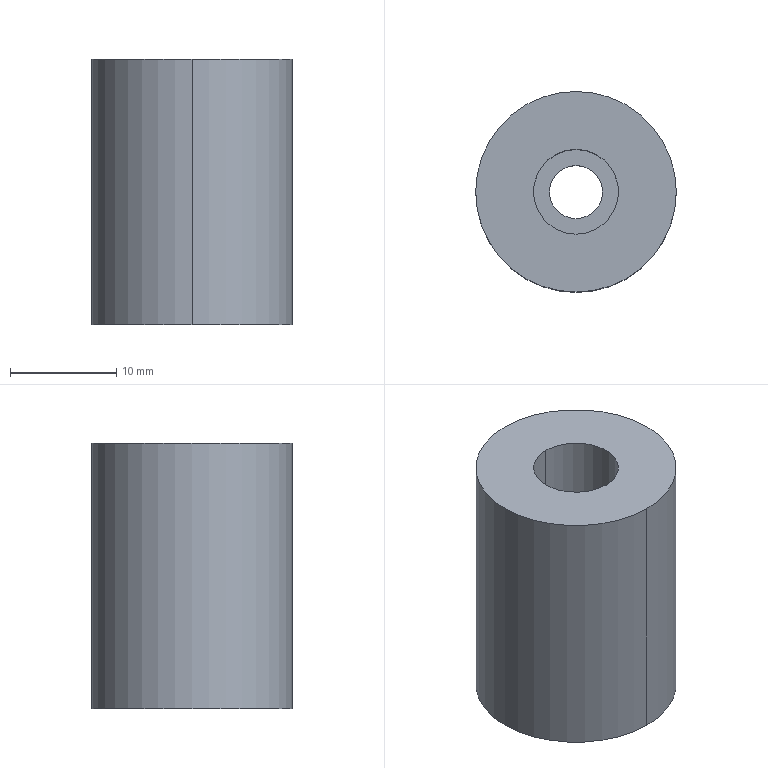Component | SolidWorks | Coupling2-1 | 1 solid | 9 faces | box 18.9 x 18.9 x 25 mm | volume 6033 mm3 | cylinder 6 | plane 3 | commonest cylinder face diameters 18.9 x2 8 x2 5 x2
STEP:
#1=COLOUR_RGB('',0.7922,0.8196,0.9333);
#2=FILL_AREA_STYLE_COLOUR('',#1);
#3=FILL_AREA_STYLE('',(#2));
#4=SURFACE_STYLE_FILL_AREA(#3);
#5=SURFACE_SIDE_STYLE('',(#4));
#6=SURFACE_STYLE_USAGE(.BOTH.,#5);
#7=PRESENTATION_STYLE_ASSIGNMENT((#6));
#8=CARTESIAN_POINT('',(0.,0.372,0.5315));
#9=VERTEX_POINT('',#8);
#10=CARTESIAN_POINT('',(-0.,-0.372,0.5315));
#11=VERTEX_POINT('',#10);
#12=CARTESIAN_POINT('',(0.,0.,0.5315));
#13=DIRECTION('',(-0.,-0.,1.));
#14=DIRECTION('',(-0.,1.,0.));
#15=AXIS2_PLACEMENT_3D('',#12,#13,#14);
#16=CIRCLE('',#15,0.372);
#17=EDGE_CURVE('',#9,#11,#16,.T.);
#18=ORIENTED_EDGE('',*,*,#17,.T.);
#19=CARTESIAN_POINT('',(-0.,-0.372,1.516));
#20=VERTEX_POINT('',#19);
#21=CARTESIAN_POINT('',(0.,-0.372,0.5315));
#22=DIRECTION('',(-0.,-0.,1.));
#23=VECTOR('',#22,39.37);
#24=LINE('',#21,#23);
#25=EDGE_CURVE('',#11,#20,#24,.T.);
#26=ORIENTED_EDGE('',*,*,#25,.T.);
#27=CARTESIAN_POINT('',(-0.,0.372,1.516));
#28=VERTEX_POINT('',#27);
#29=CARTESIAN_POINT('',(-0.,-0.,1.516));
#30=DIRECTION('',(0.,0.,-1.));
#31=DIRECTION('',(-0.,1.,0.));
#32=AXIS2_PLACEMENT_3D('',#29,#30,#31);
#33=CIRCLE('',#32,0.372);
#34=EDGE_CURVE('',#20,#28,#33,.T.);
#35=ORIENTED_EDGE('',*,*,#34,.T.);
#36=CARTESIAN_POINT('',(0.,0.372,0.5315));
#37=DIRECTION('',(-0.,-0.,1.));
#38=VECTOR('',#37,39.37);
#39=LINE('',#36,#38);
#40=EDGE_CURVE('',#9,#28,#39,.T.);
#41=ORIENTED_EDGE('',*,*,#40,.F.);
#42=EDGE_LOOP('',(#18,#26,#35,#41));
#43=FACE_OUTER_BOUND('',#42,.T.);
#44=CARTESIAN_POINT('',(0.,0.,0.5315));
#45=DIRECTION('',(-0.,-0.,1.));
#46=DIRECTION('',(-0.,1.,0.));
#47=AXIS2_PLACEMENT_3D('',#44,#45,#46);
#48=CYLINDRICAL_SURFACE('',#47,0.372);
#49=ADVANCED_FACE('',(#43),#48,.T.);
#50=CARTESIAN_POINT('',(-0.,-0.1575,0.8858));
#51=VERTEX_POINT('',#50);
#52=CARTESIAN_POINT('',(-0.,0.1575,0.8858));
#53=VERTEX_POINT('',#52);
#54=CARTESIAN_POINT('',(-0.,0.,0.8858));
#55=DIRECTION('',(-0.,-0.,1.));
#56=DIRECTION('',(-0.,1.,0.));
#57=AXIS2_PLACEMENT_3D('',#54,#55,#56);
#58=CIRCLE('',#57,0.1575);
#59=EDGE_CURVE('',#51,#53,#58,.T.);
#60=ORIENTED_EDGE('',*,*,#59,.F.);
#61=CARTESIAN_POINT('',(-0.,-0.1575,1.516));
#62=VERTEX_POINT('',#61);
#63=CARTESIAN_POINT('',(-0.,-0.1575,0.8858));
#64=DIRECTION('',(-0.,-0.,1.));
#65=VECTOR('',#64,39.37);
#66=LINE('',#63,#65);
#67=EDGE_CURVE('',#51,#62,#66,.T.);
#68=ORIENTED_EDGE('',*,*,#67,.T.);
#69=CARTESIAN_POINT('',(-0.,0.1575,1.516));
#70=VERTEX_POINT('',#69);
#71=CARTESIAN_POINT('',(-0.,-0.,1.516));
#72=DIRECTION('',(-0.,-0.,1.));
#73=DIRECTION('',(-0.,1.,0.));
#74=AXIS2_PLACEMENT_3D('',#71,#72,#73);
#75=CIRCLE('',#74,0.1575);
#76=EDGE_CURVE('',#62,#70,#75,.T.);
#77=ORIENTED_EDGE('',*,*,#76,.T.);
#78=CARTESIAN_POINT('',(-0.,0.1575,0.8858));
#79=DIRECTION('',(-0.,-0.,1.));
#80=VECTOR('',#79,39.37);
#81=LINE('',#78,#80);
#82=EDGE_CURVE('',#53,#70,#81,.T.);
#83=ORIENTED_EDGE('',*,*,#82,.F.);
#84=EDGE_LOOP('',(#60,#68,#77,#83));
#85=FACE_OUTER_BOUND('',#84,.T.);
#86=CARTESIAN_POINT('',(-0.,0.,0.8858));
#87=DIRECTION('',(-0.,-0.,1.));
#88=DIRECTION('',(-0.,1.,0.));
#89=AXIS2_PLACEMENT_3D('',#86,#87,#88);
#90=CYLINDRICAL_SURFACE('',#89,0.1575);
#91=ADVANCED_FACE('',(#85),#90,.F.);
#92=CARTESIAN_POINT('',(0.,-0.09843,0.5315));
#93=VERTEX_POINT('',#92);
#94=CARTESIAN_POINT('',(0.,0.09843,0.5315));
#95=VERTEX_POINT('',#94);
#96=CARTESIAN_POINT('',(0.,0.,0.5315));
#97=DIRECTION('',(-0.,-0.,1.));
#98=DIRECTION('',(-0.,1.,0.));
#99=AXIS2_PLACEMENT_3D('',#96,#97,#98);
#100=CIRCLE('',#99,0.09843);
#101=EDGE_CURVE('',#93,#95,#100,.T.);
#102=ORIENTED_EDGE('',*,*,#101,.F.);
#103=CARTESIAN_POINT('',(0.,-0.09843,0.8858));
#104=VERTEX_POINT('',#103);
#105=CARTESIAN_POINT('',(0.,-0.09843,0.2559));
#106=DIRECTION('',(-0.,-0.,1.));
#107=VECTOR('',#106,39.37);
#108=LINE('',#105,#107);
#109=EDGE_CURVE('',#93,#104,#108,.T.);
#110=ORIENTED_EDGE('',*,*,#109,.T.);
#111=CARTESIAN_POINT('',(-0.,0.09843,0.8858));
#112=VERTEX_POINT('',#111);
#113=CARTESIAN_POINT('',(-0.,0.,0.8858));
#114=DIRECTION('',(0.,0.,-1.));
#115=DIRECTION('',(-0.,1.,0.));
#116=AXIS2_PLACEMENT_3D('',#113,#114,#115);
#117=CIRCLE('',#116,0.09843);
#118=EDGE_CURVE('',#112,#104,#117,.T.);
#119=ORIENTED_EDGE('',*,*,#118,.F.);
#120=CARTESIAN_POINT('',(0.,0.09843,0.2559));
#121=DIRECTION('',(-0.,-0.,1.));
#122=VECTOR('',#121,39.37);
#123=LINE('',#120,#122);
#124=EDGE_CURVE('',#95,#112,#123,.T.);
#125=ORIENTED_EDGE('',*,*,#124,.F.);
#126=EDGE_LOOP('',(#102,#110,#119,#125));
#127=FACE_OUTER_BOUND('',#126,.T.);
#128=CARTESIAN_POINT('',(0.,0.,0.2559));
#129=DIRECTION('',(-0.,-0.,1.));
#130=DIRECTION('',(-0.,1.,0.));
#131=AXIS2_PLACEMENT_3D('',#128,#129,#130);
#132=CYLINDRICAL_SURFACE('',#131,0.09843);
#133=ADVANCED_FACE('',(#127),#132,.F.);
#134=ORIENTED_EDGE('',*,*,#25,.F.);
#135=CARTESIAN_POINT('',(0.,0.,0.5315));
#136=DIRECTION('',(-0.,-0.,1.));
#137=DIRECTION('',(-0.,1.,0.));
#138=AXIS2_PLACEMENT_3D('',#135,#136,#137);
#139=CIRCLE('',#138,0.372);
#140=EDGE_CURVE('',#11,#9,#139,.T.);
#141=ORIENTED_EDGE('',*,*,#140,.T.);
#142=ORIENTED_EDGE('',*,*,#40,.T.);
#143=CARTESIAN_POINT('',(-0.,-0.,1.516));
#144=DIRECTION('',(0.,0.,-1.));
#145=DIRECTION('',(-0.,1.,0.));
#146=AXIS2_PLACEMENT_3D('',#143,#144,#145);
#147=CIRCLE('',#146,0.372);
#148=EDGE_CURVE('',#28,#20,#147,.T.);
#149=ORIENTED_EDGE('',*,*,#148,.T.);
#150=EDGE_LOOP('',(#134,#141,#142,#149));
#151=FACE_OUTER_BOUND('',#150,.T.);
#152=CARTESIAN_POINT('',(0.,0.,0.5315));
#153=DIRECTION('',(-0.,-0.,1.));
#154=DIRECTION('',(-0.,1.,0.));
#155=AXIS2_PLACEMENT_3D('',#152,#153,#154);
#156=CYLINDRICAL_SURFACE('',#155,0.372);
#157=ADVANCED_FACE('',(#151),#156,.T.);
#158=ORIENTED_EDGE('',*,*,#148,.F.);
#159=ORIENTED_EDGE('',*,*,#34,.F.);
#160=EDGE_LOOP('',(#158,#159));
#161=FACE_OUTER_BOUND('',#160,.T.);
#162=CARTESIAN_POINT('',(-0.,-0.,1.516));
#163=DIRECTION('',(-0.,-0.,1.));
#164=DIRECTION('',(-0.,1.,0.));
#165=AXIS2_PLACEMENT_3D('',#162,#163,#164);
#166=CIRCLE('',#165,0.1575);
#167=EDGE_CURVE('',#70,#62,#166,.T.);
#168=ORIENTED_EDGE('',*,*,#167,.F.);
#169=ORIENTED_EDGE('',*,*,#76,.F.);
#170=EDGE_LOOP('',(#168,#169));
#171=FACE_BOUND('',#170,.T.);
#172=CARTESIAN_POINT('',(-0.,-0.,1.516));
#173=DIRECTION('',(0.,0.,-1.));
#174=DIRECTION('',(0.,-1.,-0.));
#175=AXIS2_PLACEMENT_3D('',#172,#173,#174);
#176=PLANE('',#175);
#177=ADVANCED_FACE('',(#161,#171),#176,.F.);
#178=ORIENTED_EDGE('',*,*,#17,.F.);
#179=ORIENTED_EDGE('',*,*,#140,.F.);
#180=EDGE_LOOP('',(#178,#179));
#181=FACE_OUTER_BOUND('',#180,.T.);
#182=CARTESIAN_POINT('',(0.,0.,0.5315));
#183=DIRECTION('',(-0.,-0.,1.));
#184=DIRECTION('',(-0.,1.,0.));
#185=AXIS2_PLACEMENT_3D('',#182,#183,#184);
#186=CIRCLE('',#185,0.09843);
#187=EDGE_CURVE('',#95,#93,#186,.T.);
#188=ORIENTED_EDGE('',*,*,#187,.T.);
#189=ORIENTED_EDGE('',*,*,#101,.T.);
#190=EDGE_LOOP('',(#188,#189));
#191=FACE_BOUND('',#190,.T.);
#192=CARTESIAN_POINT('',(0.,0.,0.5315));
#193=DIRECTION('',(0.,0.,-1.));
#194=DIRECTION('',(0.,-1.,-0.));
#195=AXIS2_PLACEMENT_3D('',#192,#193,#194);
#196=PLANE('',#195);
#197=ADVANCED_FACE('',(#181,#191),#196,.T.);
#198=ORIENTED_EDGE('',*,*,#67,.F.);
#199=CARTESIAN_POINT('',(-0.,0.,0.8858));
#200=DIRECTION('',(-0.,-0.,1.));
#201=DIRECTION('',(-0.,1.,0.));
#202=AXIS2_PLACEMENT_3D('',#199,#200,#201);
#203=CIRCLE('',#202,0.1575);
#204=EDGE_CURVE('',#53,#51,#203,.T.);
#205=ORIENTED_EDGE('',*,*,#204,.F.);
#206=ORIENTED_EDGE('',*,*,#82,.T.);
#207=ORIENTED_EDGE('',*,*,#167,.T.);
#208=EDGE_LOOP('',(#198,#205,#206,#207));
#209=FACE_OUTER_BOUND('',#208,.T.);
#210=CARTESIAN_POINT('',(-0.,0.,0.8858));
#211=DIRECTION('',(-0.,-0.,1.));
#212=DIRECTION('',(-0.,1.,0.));
#213=AXIS2_PLACEMENT_3D('',#210,#211,#212);
#214=CYLINDRICAL_SURFACE('',#213,0.1575);
#215=ADVANCED_FACE('',(#209),#214,.F.);
#216=ORIENTED_EDGE('',*,*,#109,.F.);
#217=ORIENTED_EDGE('',*,*,#187,.F.);
#218=ORIENTED_EDGE('',*,*,#124,.T.);
#219=CARTESIAN_POINT('',(-0.,0.,0.8858));
#220=DIRECTION('',(0.,0.,-1.));
#221=DIRECTION('',(-0.,1.,0.));
#222=AXIS2_PLACEMENT_3D('',#219,#220,#221);
#223=CIRCLE('',#222,0.09843);
#224=EDGE_CURVE('',#104,#112,#223,.T.);
#225=ORIENTED_EDGE('',*,*,#224,.F.);
#226=EDGE_LOOP('',(#216,#217,#218,#225));
#227=FACE_OUTER_BOUND('',#226,.T.);
#228=CARTESIAN_POINT('',(0.,0.,0.2559));
#229=DIRECTION('',(-0.,-0.,1.));
#230=DIRECTION('',(-0.,1.,0.));
#231=AXIS2_PLACEMENT_3D('',#228,#229,#230);
#232=CYLINDRICAL_SURFACE('',#231,0.09843);
#233=ADVANCED_FACE('',(#227),#232,.F.);
#234=ORIENTED_EDGE('',*,*,#204,.T.);
#235=ORIENTED_EDGE('',*,*,#59,.T.);
#236=EDGE_LOOP('',(#234,#235));
#237=FACE_OUTER_BOUND('',#236,.T.);
#238=ORIENTED_EDGE('',*,*,#118,.T.);
#239=ORIENTED_EDGE('',*,*,#224,.T.);
#240=EDGE_LOOP('',(#238,#239));
#241=FACE_BOUND('',#240,.T.);
#242=CARTESIAN_POINT('',(-0.,0.,0.8858));
#243=DIRECTION('',(-0.,-0.,1.));
#244=DIRECTION('',(-0.,1.,0.));
#245=AXIS2_PLACEMENT_3D('',#242,#243,#244);
#246=PLANE('',#245);
#247=ADVANCED_FACE('',(#237,#241),#246,.T.);
#248=CLOSED_SHELL('',(#49,#91,#133,#157,#177,#197,#215,#233,#247));
#249=MANIFOLD_SOLID_BREP('',#248);
#250=STYLED_ITEM('',(#7),#249);
#251=PRESENTATION_LAYER_ASSIGNMENT('','',(#250));
#252=(LENGTH_UNIT()NAMED_UNIT(*)SI_UNIT($,.METRE.));
#253=LENGTH_MEASURE_WITH_UNIT(LENGTH_MEASURE(0.0254),#252);
#254=DIMENSIONAL_EXPONENTS(1.,0.,0.,0.,0.,0.,0.);
#255=(CONVERSION_BASED_UNIT('',#253)LENGTH_UNIT()NAMED_UNIT(#254));
#256=UNCERTAINTY_MEASURE_WITH_UNIT(LENGTH_MEASURE(0.00001),#255,'','');
#257=(NAMED_UNIT(*)PLANE_ANGLE_UNIT()SI_UNIT($,.RADIAN.));
#258=(NAMED_UNIT(*)SI_UNIT($,.STERADIAN.)SOLID_ANGLE_UNIT());
#259=(GEOMETRIC_REPRESENTATION_CONTEXT(3)GLOBAL_UNCERTAINTY_ASSIGNED_CONTEXT((#256))GLOBAL_UNIT_ASSIGNED_CONTEXT((#255,#257,#258))REPRESENTATION_CONTEXT('',''));
#260=MECHANICAL_DESIGN_GEOMETRIC_PRESENTATION_REPRESENTATION('',(#250),#259);
#261=CARTESIAN_POINT('',(0.,0.,0.));
#262=DIRECTION('',(0.,0.,1.));
#263=DIRECTION('',(1.,0.,0.));
#264=AXIS2_PLACEMENT_3D('',#261,#262,#263);
#265=(LENGTH_UNIT()NAMED_UNIT(*)SI_UNIT($,.METRE.));
#266=LENGTH_MEASURE_WITH_UNIT(LENGTH_MEASURE(0.0254),#265);
#267=DIMENSIONAL_EXPONENTS(1.,0.,0.,0.,0.,0.,0.);
#268=(CONVERSION_BASED_UNIT('',#266)LENGTH_UNIT()NAMED_UNIT(#267));
#269=UNCERTAINTY_MEASURE_WITH_UNIT(LENGTH_MEASURE(0.00001),#268,'','');
#270=(NAMED_UNIT(*)PLANE_ANGLE_UNIT()SI_UNIT($,.RADIAN.));
#271=(NAMED_UNIT(*)SI_UNIT($,.STERADIAN.)SOLID_ANGLE_UNIT());
#272=(GEOMETRIC_REPRESENTATION_CONTEXT(3)GLOBAL_UNCERTAINTY_ASSIGNED_CONTEXT((#269))GLOBAL_UNIT_ASSIGNED_CONTEXT((#268,#270,#271))REPRESENTATION_CONTEXT('',''));
#273=ADVANCED_BREP_SHAPE_REPRESENTATION('',(#249,#264),#272);